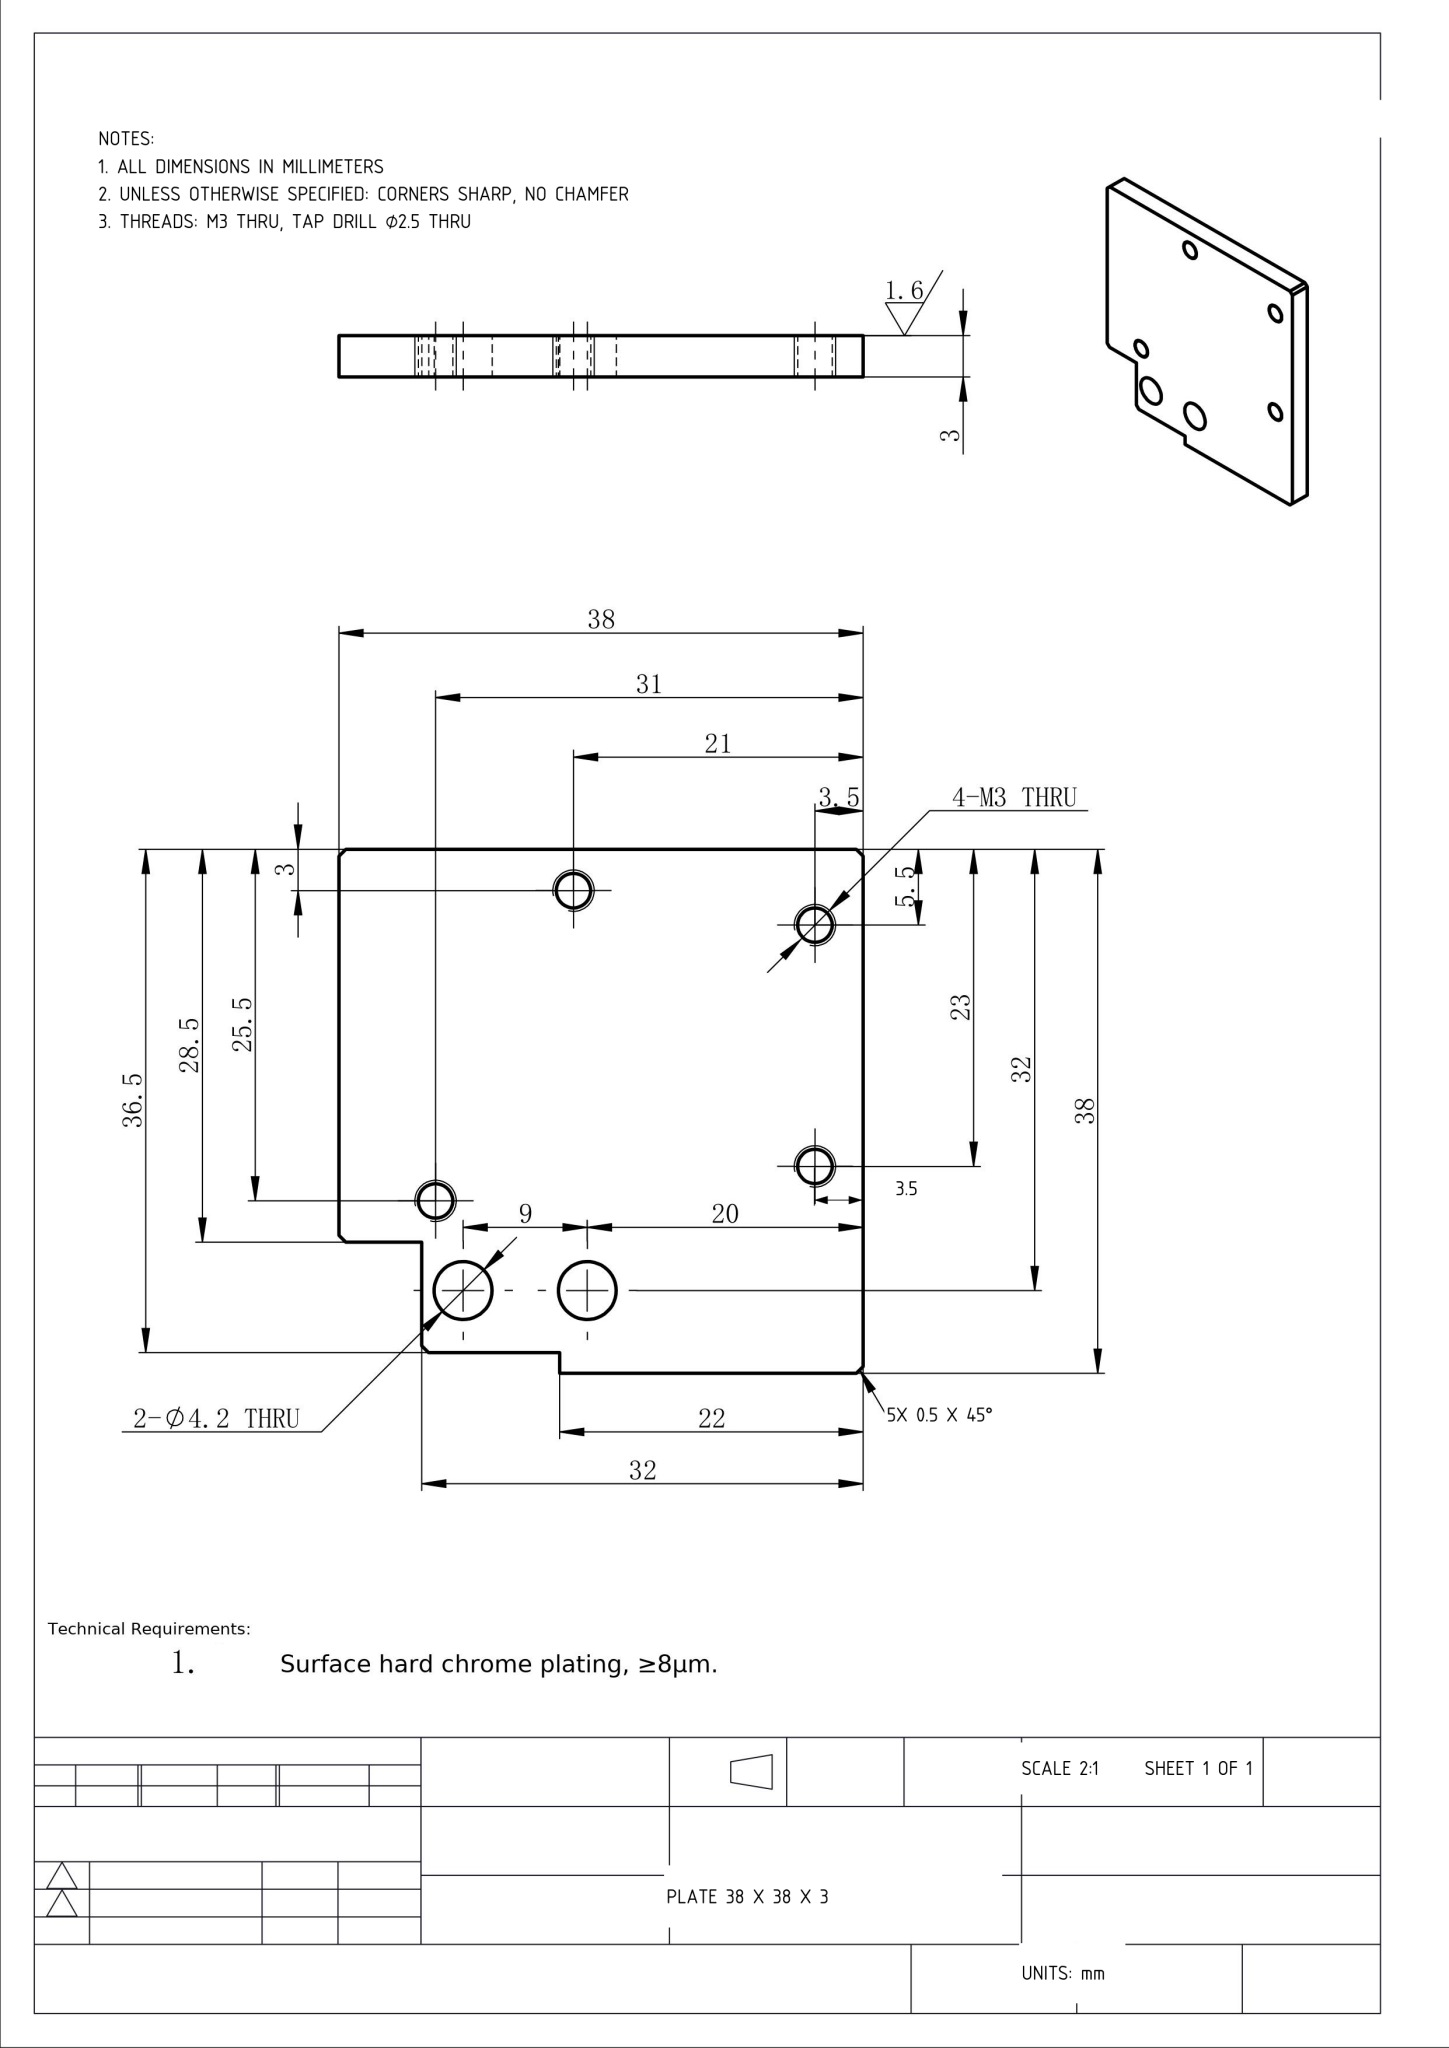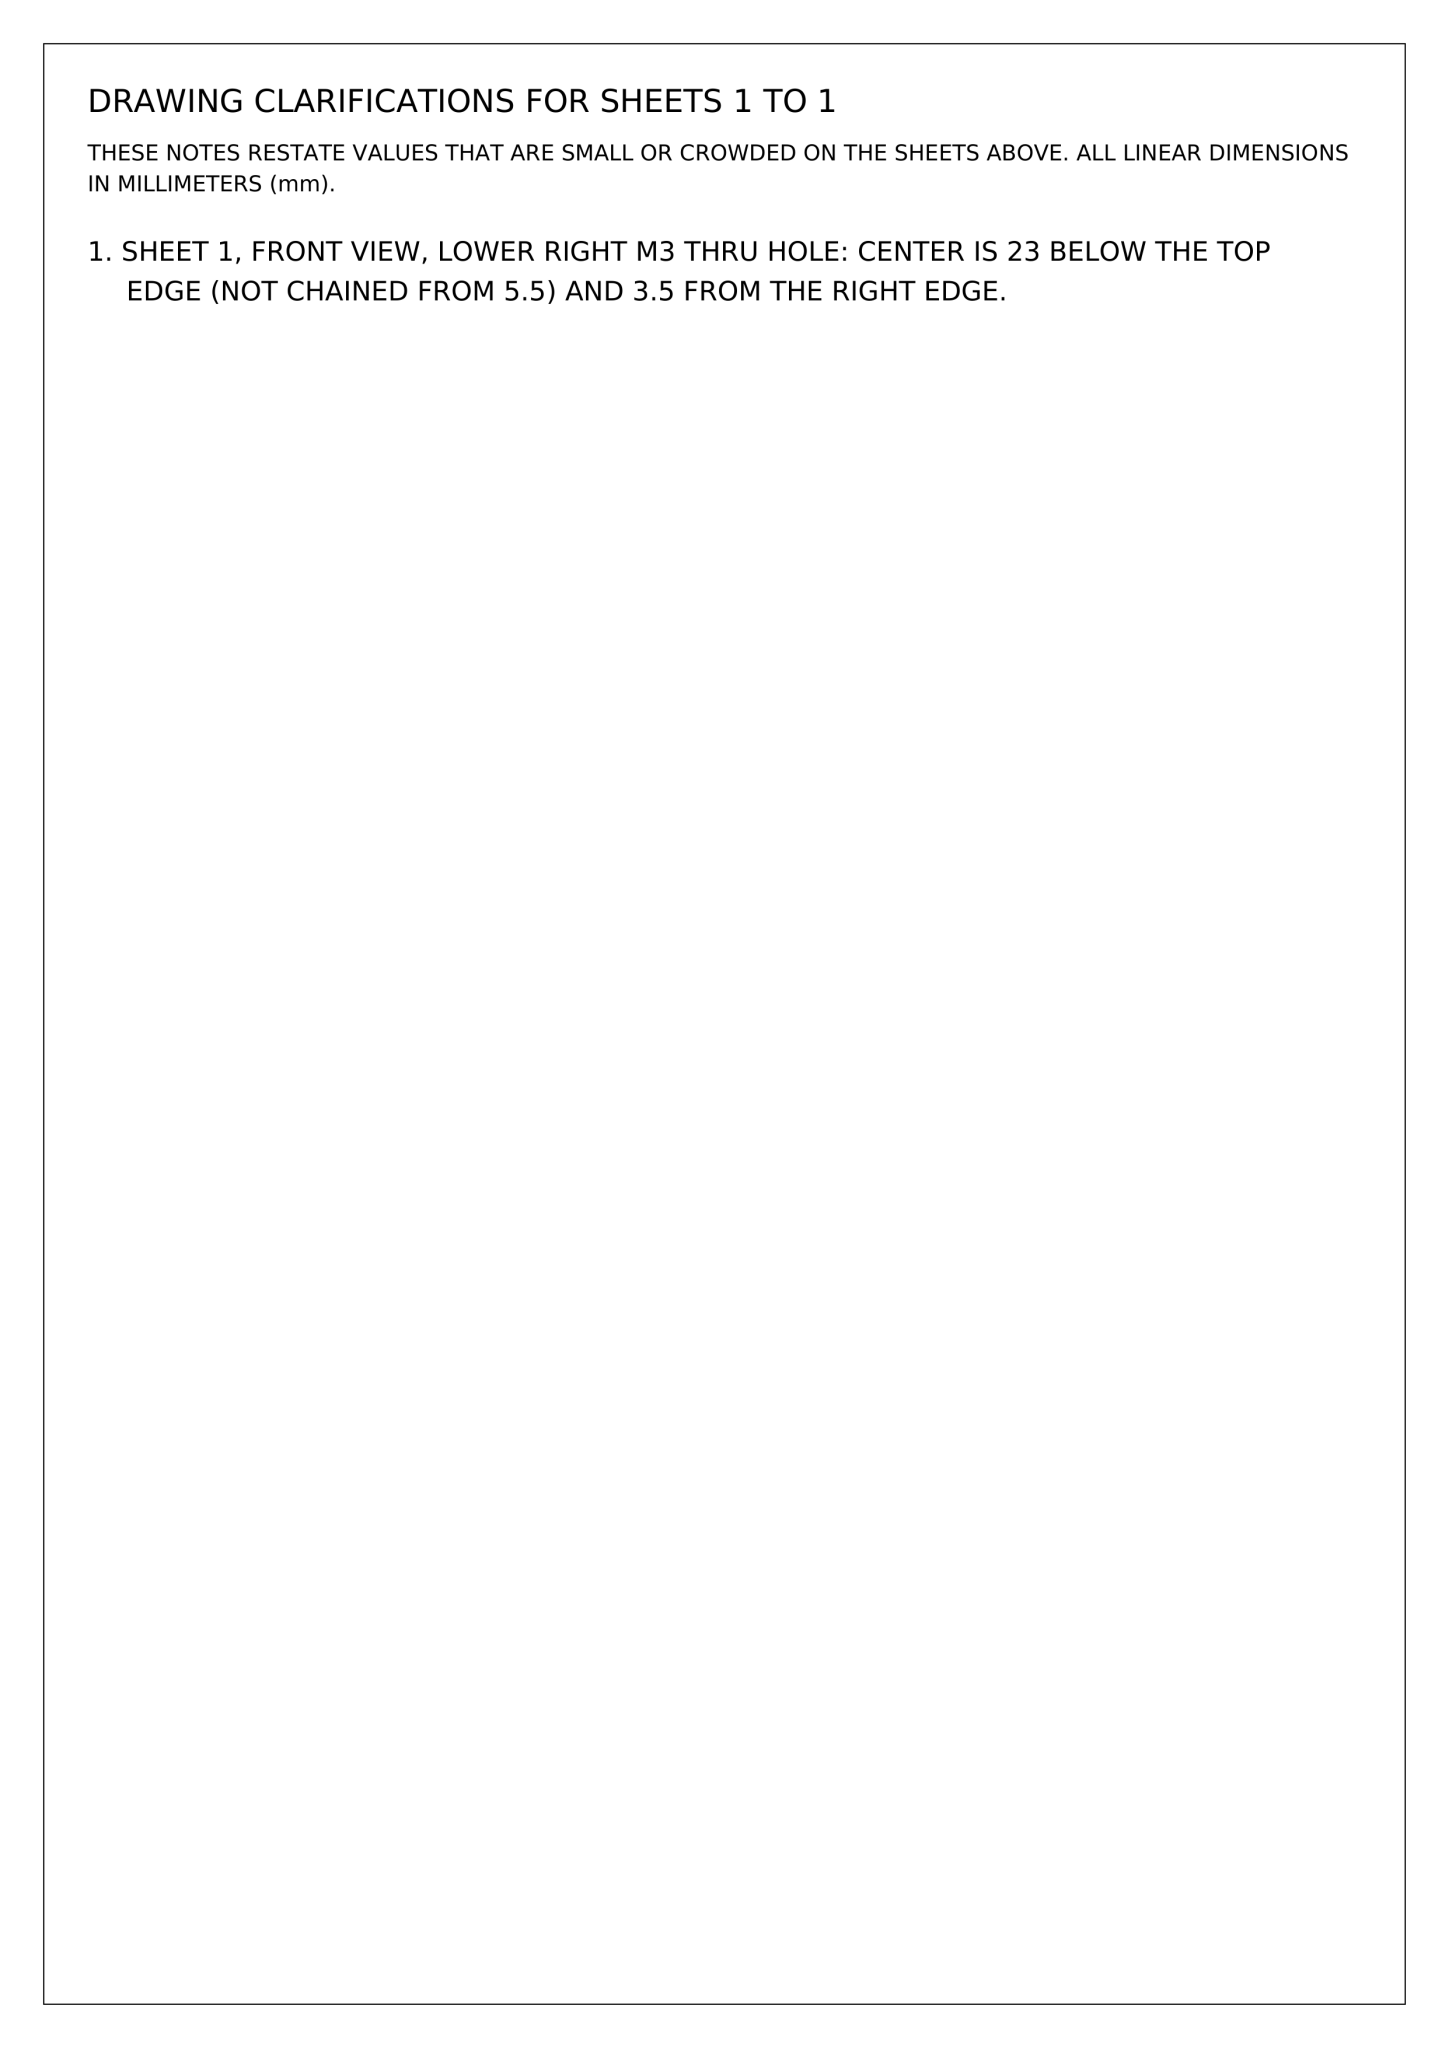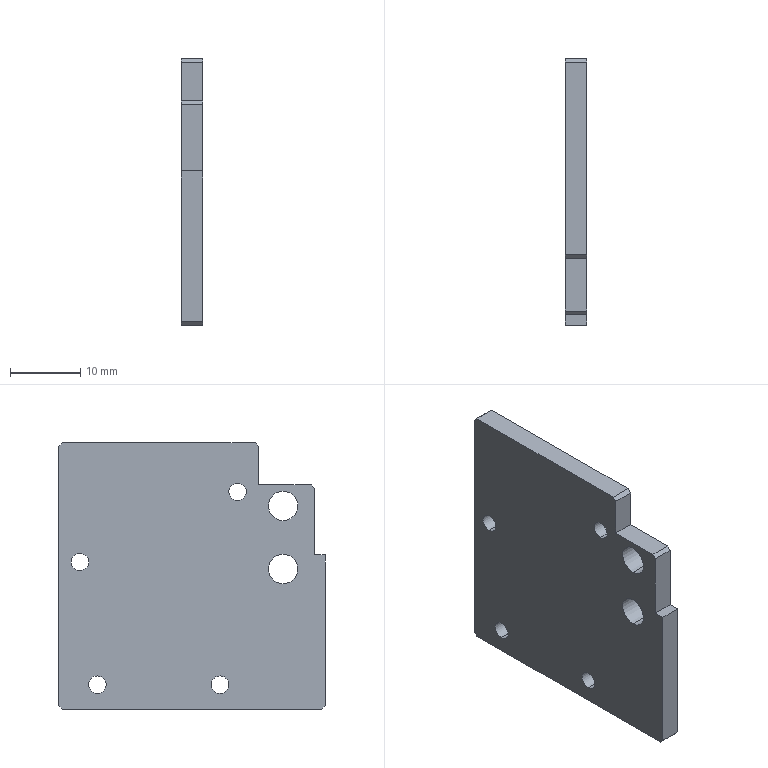Part | NX | mm | Stepped Edge Multi-Bore Mounting Plate | 1 solid | 27 faces | box 3 x 38 x 38 mm | volume 3972 mm3 | plane 15 | cylinder 12 | commonest cylinder face diameters 2.5 x8 4.2 x4